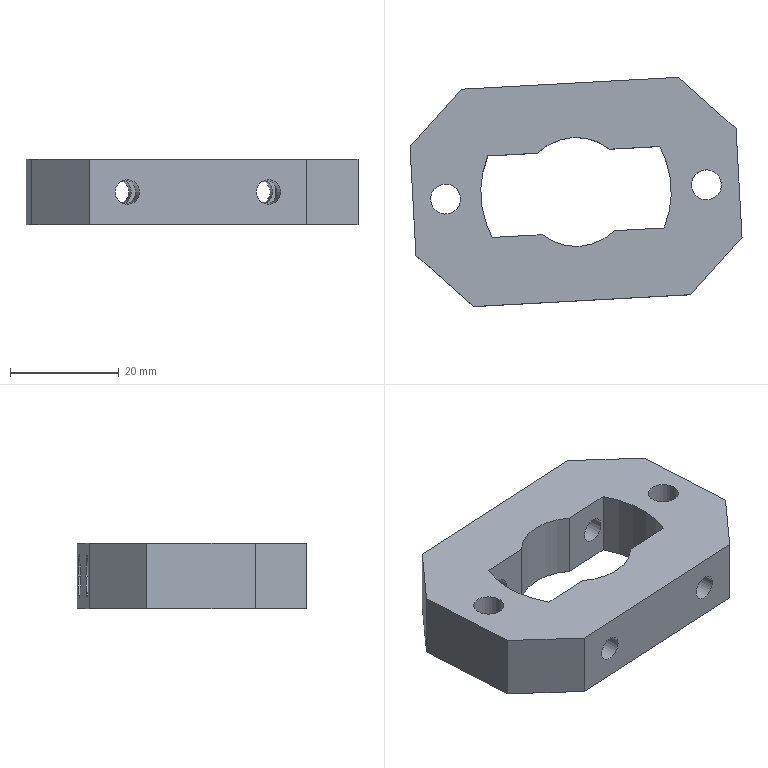Component | SolidWorks | BearingPressPartM-1 | 1 solid | 43 faces | box 61 x 42.13 x 12 mm | volume 17486 mm3 | cylinder 25 | plane 18 | commonest cylinder face diameters 4.5 x8 10 x4 5.5 x4 8 x4 20.05 x3 35 x2
build123d program:
from build123d import *

# Parameters (mm, degrees)
SKETCH1_W                                       = 12
SKETCH1_H                                       = 40
BOSS_EXTRUDE1_DEPTH                             = 60
CUT_EXTRUDE1_DEPTH                              = 65.753
CHAMFER1_SIZE                                   = 10
M4_HEX_SOCKET_HEAD_CAP_SCREW_CBORE1_D           = 4.5
M4_HEX_SOCKET_HEAD_CAP_SCREW_CBORE1_CBORE_D     = 8
M4_HEX_SOCKET_HEAD_CAP_SCREW_CBORE1_CBORE_DEPTH = 4.4
M5_HEX_SOCKET_HEAD_CAP_SCREW_CBORE1_D           = 5.5
M5_HEX_SOCKET_HEAD_CAP_SCREW_CBORE1_DEPTH       = 14
M5_HEX_SOCKET_HEAD_CAP_SCREW_CBORE1_CBORE_D     = 10
M5_HEX_SOCKET_HEAD_CAP_SCREW_CBORE1_CBORE_DEPTH = 5.4
M5_HEX_SOCKET_HEAD_CAP_SCREW_CBORE1_TIP         = 1.652


with BuildPart() as part:
    # Sketch1 → Boss-Extrude1 (new body)
    with BuildSketch(Plane.XY):
        with Locations((6, 1.189)):
            Rectangle(SKETCH1_W, SKETCH1_H)
    extrude(amount=BOSS_EXTRUDE1_DEPTH)

    # Sketch2 → Cut-Extrude1 (cut, through all)
    with BuildSketch(Plane.ZY):
        with BuildLine():
            Line((14.189, 8.689), (23.348, 8.689))
            ThreePointArc((23.348, 8.689), (30, 11.214), (36.652, 8.689))
            Line((36.652, 8.689), (45.811, 8.689))
            ThreePointArc((45.811, 8.689), (47.5, 1.189), (45.811, -6.311))
            Line((45.811, -6.311), (36.652, -6.311))
            ThreePointArc((36.652, -6.311), (30, -8.836), (23.348, -6.311))
            Line((23.348, -6.311), (14.189, -6.311))
            ThreePointArc((14.189, -6.311), (12.5, 1.189), (14.189, 8.689))
        make_face()
    extrude(amount=-CUT_EXTRUDE1_DEPTH, mode=Mode.SUBTRACT)

    # Chamfer1
    chamfer1_edges = [part.edges().sort_by_distance(p)[0] for p in [
        (6, -18.811, 60),
        (6, 21.189, 60),
        (6, -18.811, 0),
        (6, 21.189, 0),
    ]]
    chamfer(chamfer1_edges, length=CHAMFER1_SIZE)

    # M4 Hex Socket Head Cap Screw CBORE1 (through all)
    with Locations(Plane(origin=(0, 21.189, 0), x_dir=(1, 0, 0), z_dir=(0, 1, 0))):
        with Locations((6, -17), (6, -43)):
            CounterBoreHole(M4_HEX_SOCKET_HEAD_CAP_SCREW_CBORE1_D / 2, M4_HEX_SOCKET_HEAD_CAP_SCREW_CBORE1_CBORE_D / 2, M4_HEX_SOCKET_HEAD_CAP_SCREW_CBORE1_CBORE_DEPTH)

    # M5 Hex Socket Head Cap Screw CBORE1
    with Locations(Plane(origin=(12, 0, 0), x_dir=(0, 0, -1), z_dir=(1, 0, 0))):
        with Locations((-54, 1.189), (-6, 1.189)):
            CounterBoreHole(M5_HEX_SOCKET_HEAD_CAP_SCREW_CBORE1_D / 2, M5_HEX_SOCKET_HEAD_CAP_SCREW_CBORE1_CBORE_D / 2, M5_HEX_SOCKET_HEAD_CAP_SCREW_CBORE1_CBORE_DEPTH, depth=M5_HEX_SOCKET_HEAD_CAP_SCREW_CBORE1_DEPTH)
            with Locations((0, 0, -(M5_HEX_SOCKET_HEAD_CAP_SCREW_CBORE1_DEPTH + M5_HEX_SOCKET_HEAD_CAP_SCREW_CBORE1_TIP / 2))):  # 118° drill point
                Cone(0, M5_HEX_SOCKET_HEAD_CAP_SCREW_CBORE1_D / 2, M5_HEX_SOCKET_HEAD_CAP_SCREW_CBORE1_TIP, mode=Mode.SUBTRACT)


solid = part.part

# Placed as in the assembly
solid = solid.moved(Location((417.786, 125.136, -283.818), (-90, 86.863, 90)))